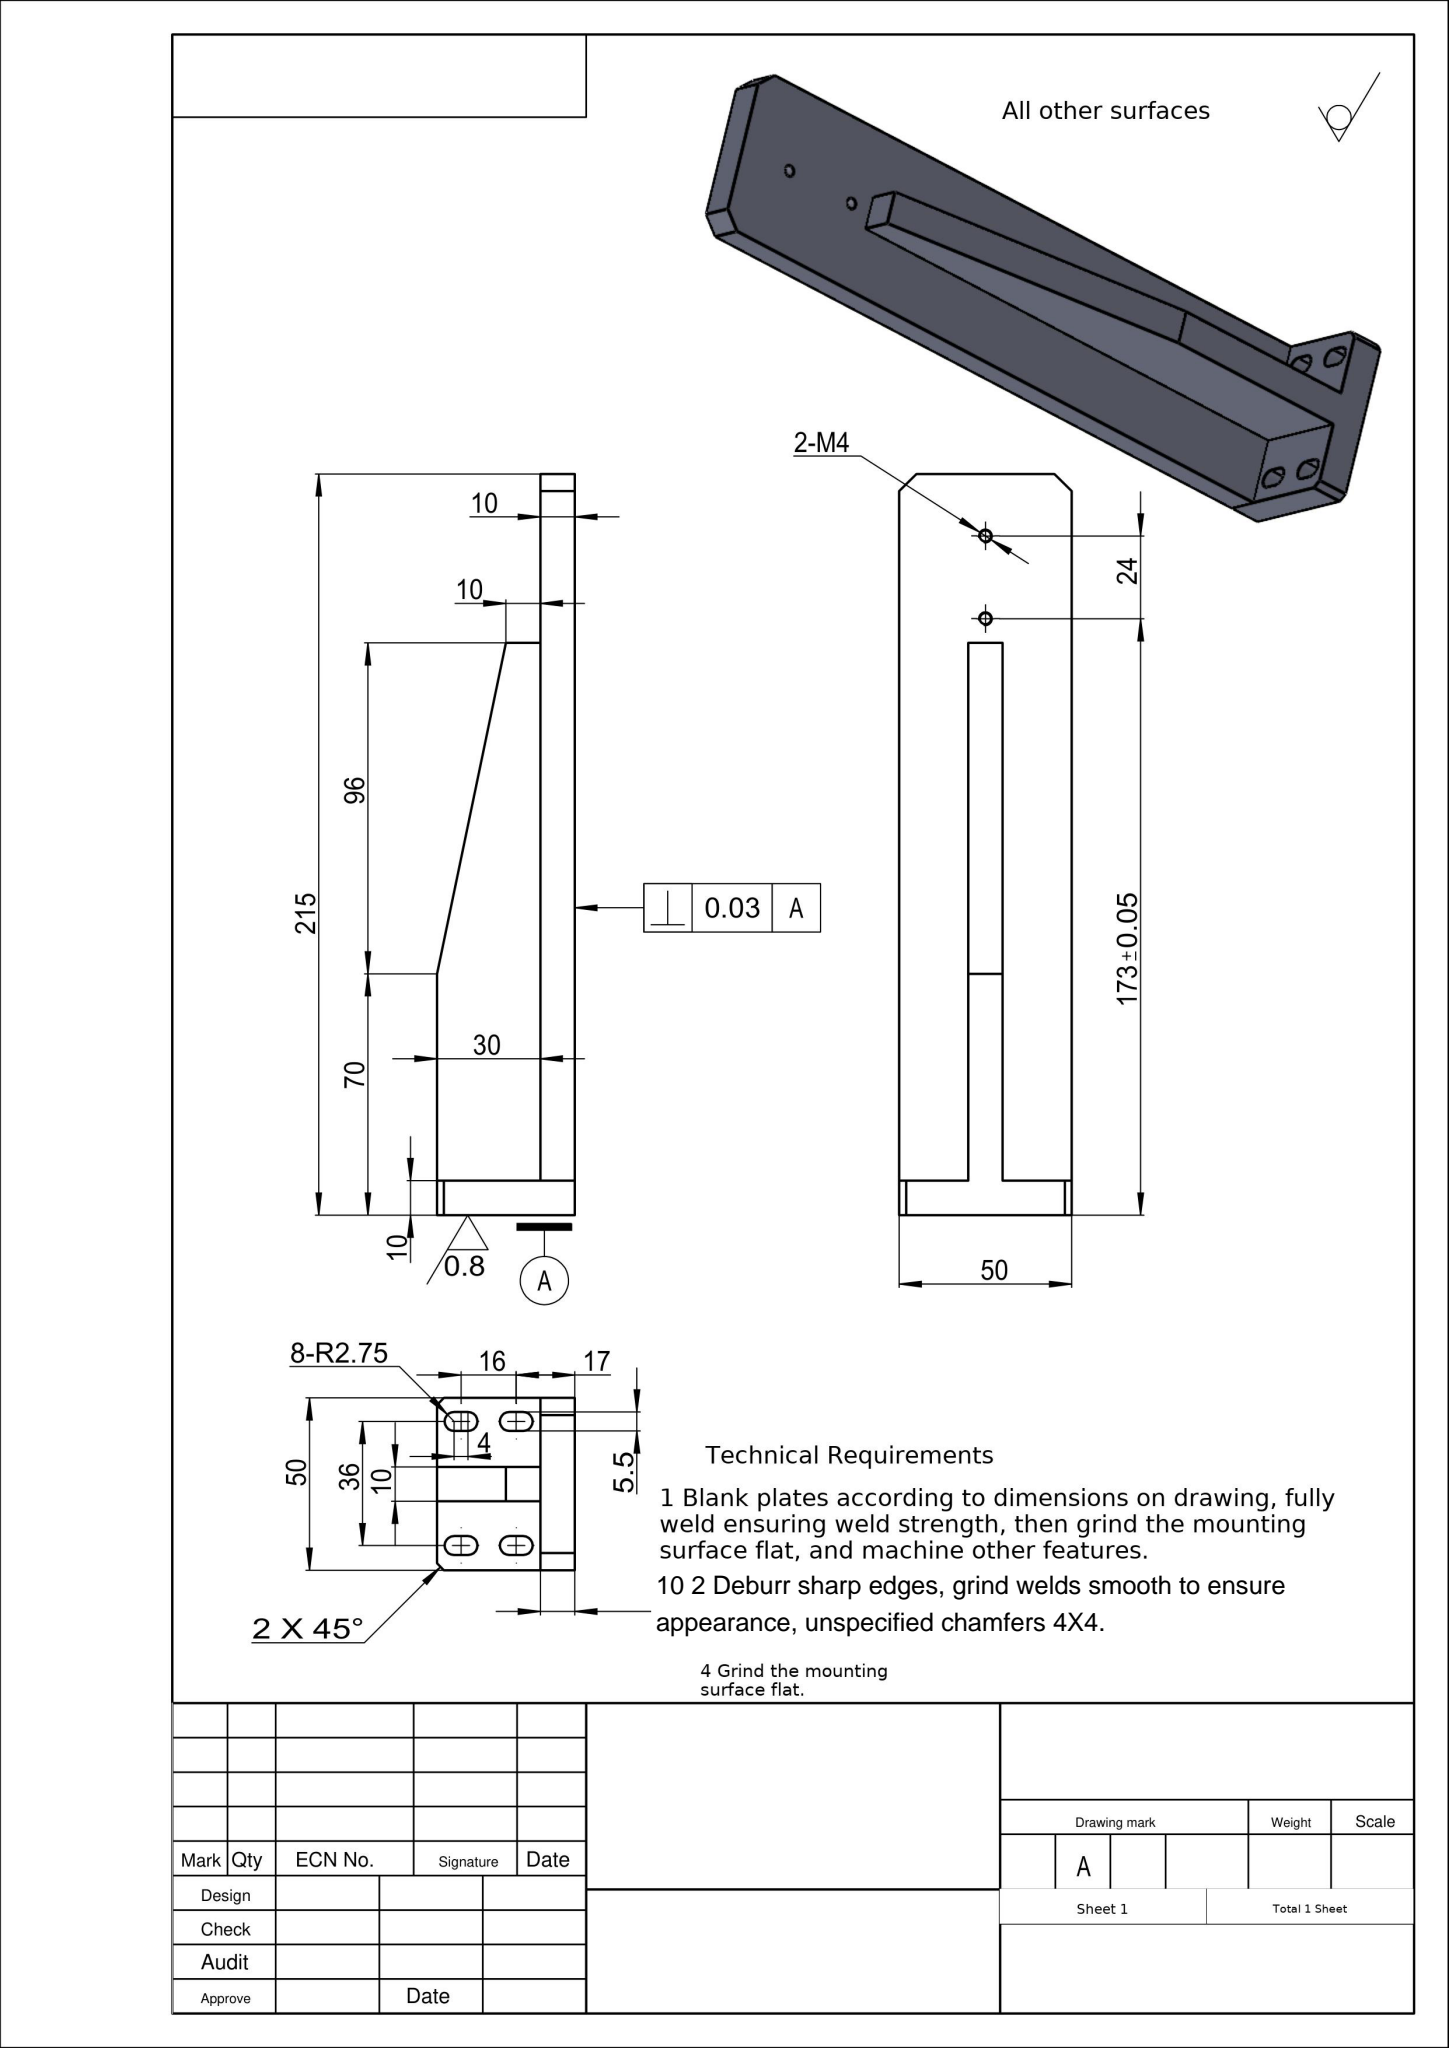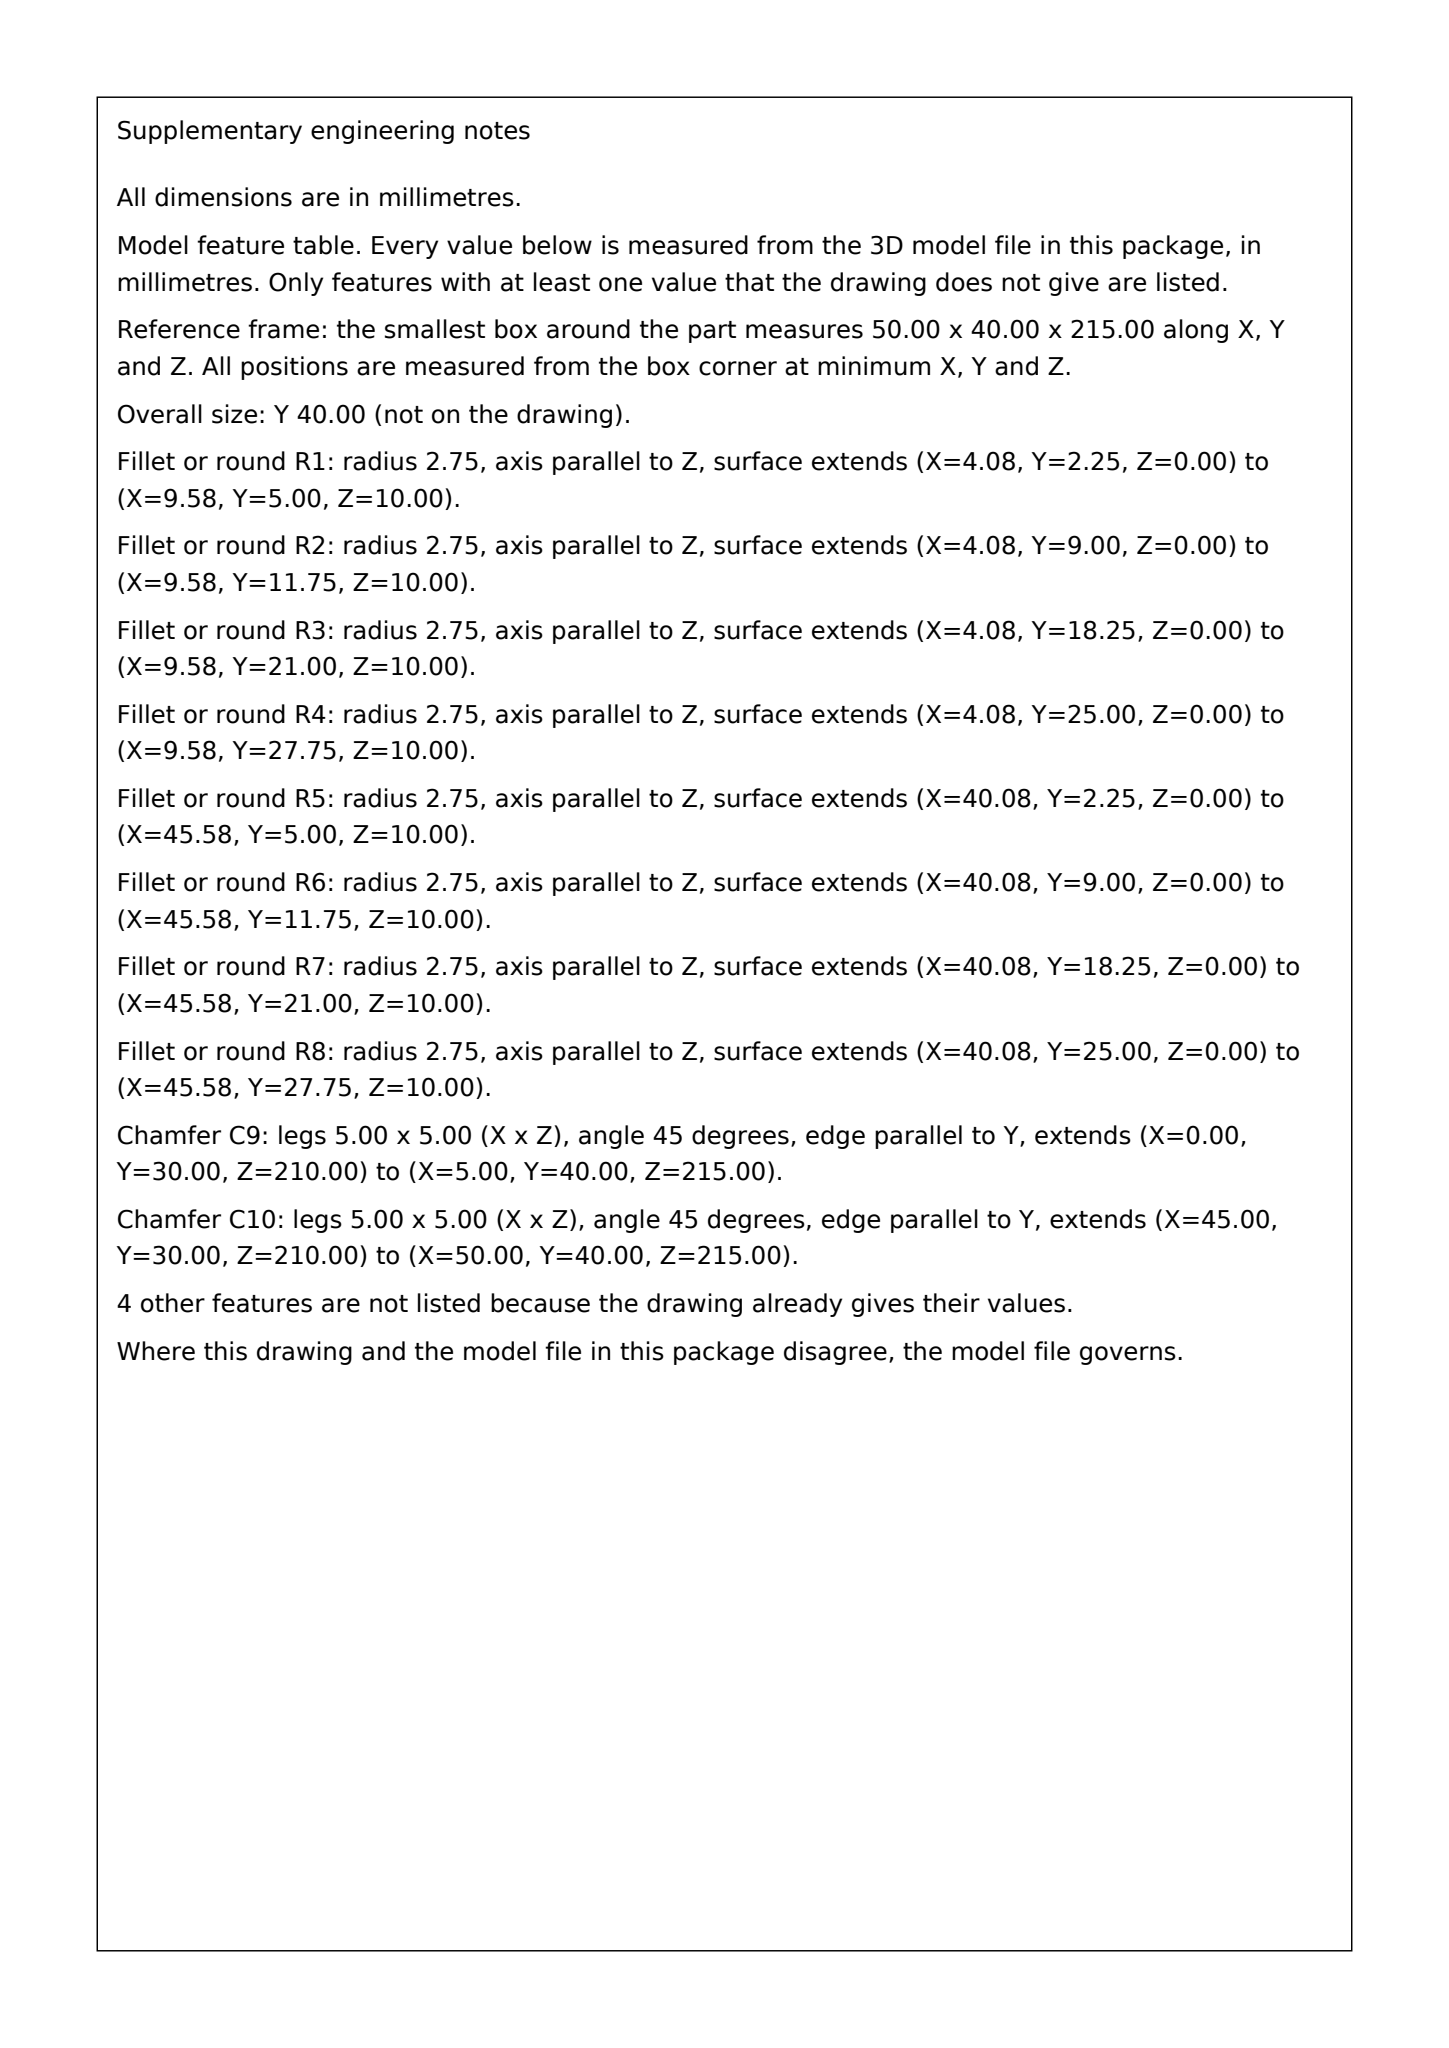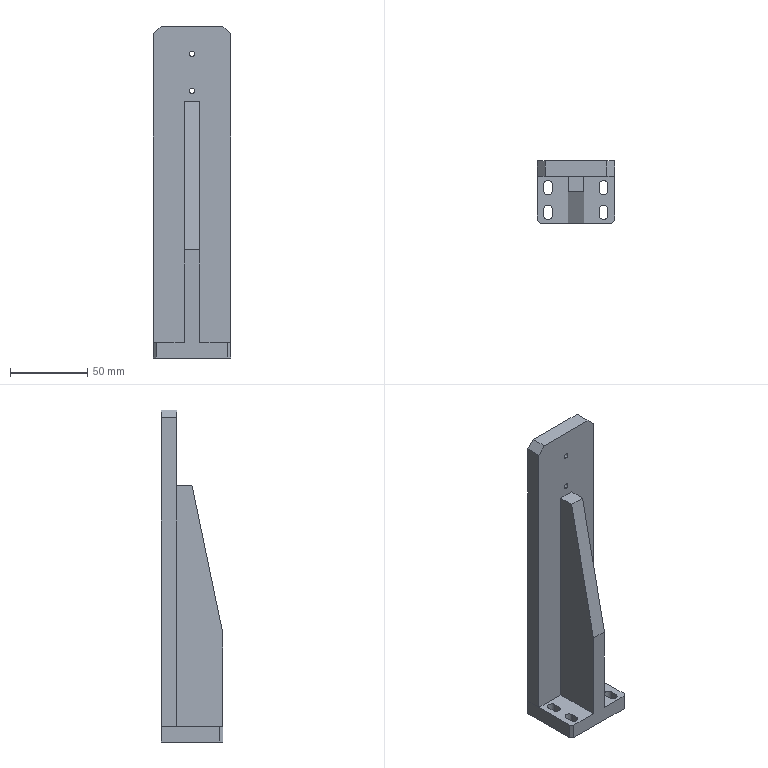Part | SolidWorks | mm | 1 solid | 39 faces | box 50 x 40 x 215 mm | volume 157408 mm3 | plane 27 | cylinder 12 | commonest cylinder face diameters 5.5 x8 3.3 x4
build123d program:
from build123d import *

# Parameters (mm, degrees)
SKETCH1_W           = 50
SKETCH1_H           = 40
BOSS_EXTRUDE1_DEPTH = 10
SKETCH2_W           = 50
SKETCH2_H           = 10
BOSS_EXTRUDE2_DEPTH = 205
SKETCH3_W           = 10
SKETCH3_H           = 30
BOSS_EXTRUDE3_DEPTH = 156
CHAMFER1_SIZE       = 96
CHAMFER1_SIZE2      = 20
CUT_EXTRUDE1_DEPTH  = 215.767
CHAMFER3_SIZE       = 2
M4_TAPPED_HOLE1_D   = 3.3
CHAMFER4_SIZE       = 5


with BuildPart() as part:
    # Sketch1 → Boss-Extrude1 (new body)
    with BuildSketch(Plane.XY):
        with Locations((25, -20)):
            Rectangle(SKETCH1_W, SKETCH1_H)
    extrude(amount=BOSS_EXTRUDE1_DEPTH)

    # Sketch2 → Boss-Extrude2 (add)
    with BuildSketch(Plane.XY.offset(10)):
        with Locations((25, -5)):
            Rectangle(SKETCH2_W, SKETCH2_H)
    extrude(amount=BOSS_EXTRUDE2_DEPTH)

    # Sketch3 → Boss-Extrude3 (add)
    with BuildSketch(Plane.XY.offset(10)):
        with Locations((25, -25)):
            Rectangle(SKETCH3_W, SKETCH3_H)
    extrude(amount=BOSS_EXTRUDE3_DEPTH)

    # Chamfer1
    chamfer1_edges = [part.edges().sort_by_distance(p)[0] for p in [
        (25, -40, 166),
    ]]
    chamfer1_side = [part.faces().sort_by_distance(p)[0] for p in [
        (25, -40, 67.854),
    ]]
    chamfer(chamfer1_edges, length=CHAMFER1_SIZE, length2=CHAMFER1_SIZE2, reference=chamfer1_side[0])

    # Sketch4 → Cut-Extrude1 (cut, through all)
    with BuildSketch(Plane.XY.offset(10)):
        with BuildLine():
            Line((9.58, -15), (9.58, -19))
            ThreePointArc((9.58, -19), (6.83, -21.75), (4.08, -19))
            Line((4.08, -19), (4.08, -15))
            ThreePointArc((4.08, -15), (6.83, -12.25), (9.58, -15))
        make_face()
        with BuildLine():
            Line((4.08, -35), (4.08, -31))
            ThreePointArc((4.08, -31), (6.83, -28.25), (9.58, -31))
            Line((9.58, -31), (9.58, -35))
            ThreePointArc((9.58, -35), (6.83, -37.75), (4.08, -35))
        make_face()
        with BuildLine():
            Line((45.58, -35), (45.58, -31))
            ThreePointArc((45.58, -31), (42.83, -28.25), (40.08, -31))
            Line((40.08, -31), (40.08, -35))
            ThreePointArc((40.08, -35), (42.83, -37.75), (45.58, -35))
        make_face()
        with BuildLine():
            Line((40.08, -15), (40.08, -19))
            ThreePointArc((40.08, -19), (42.83, -21.75), (45.58, -19))
            Line((45.58, -19), (45.58, -15))
            ThreePointArc((45.58, -15), (42.83, -12.25), (40.08, -15))
        make_face()
    extrude(amount=-CUT_EXTRUDE1_DEPTH, mode=Mode.SUBTRACT)

    # Chamfer3
    chamfer3_edges = [part.edges().sort_by_distance(p)[0] for p in [
        (50, -40, 5),
        (0, -40, 5),
    ]]
    chamfer(chamfer3_edges, length=CHAMFER3_SIZE)

    # M4 Tapped Hole1 (through all)
    with Locations(Plane(origin=(0, -0.0001, 0), x_dir=(-1, 0, 0), z_dir=(0, 1, 0))):
        with Locations((-25, 197), (-25, 173)):
            Hole(M4_TAPPED_HOLE1_D / 2)

    # Chamfer4
    chamfer4_edges = [part.edges().sort_by_distance(p)[0] for p in [
        (0.0001, -5, 215),
        (50, -5, 215),
    ]]
    chamfer(chamfer4_edges, length=CHAMFER4_SIZE)


solid = part.part